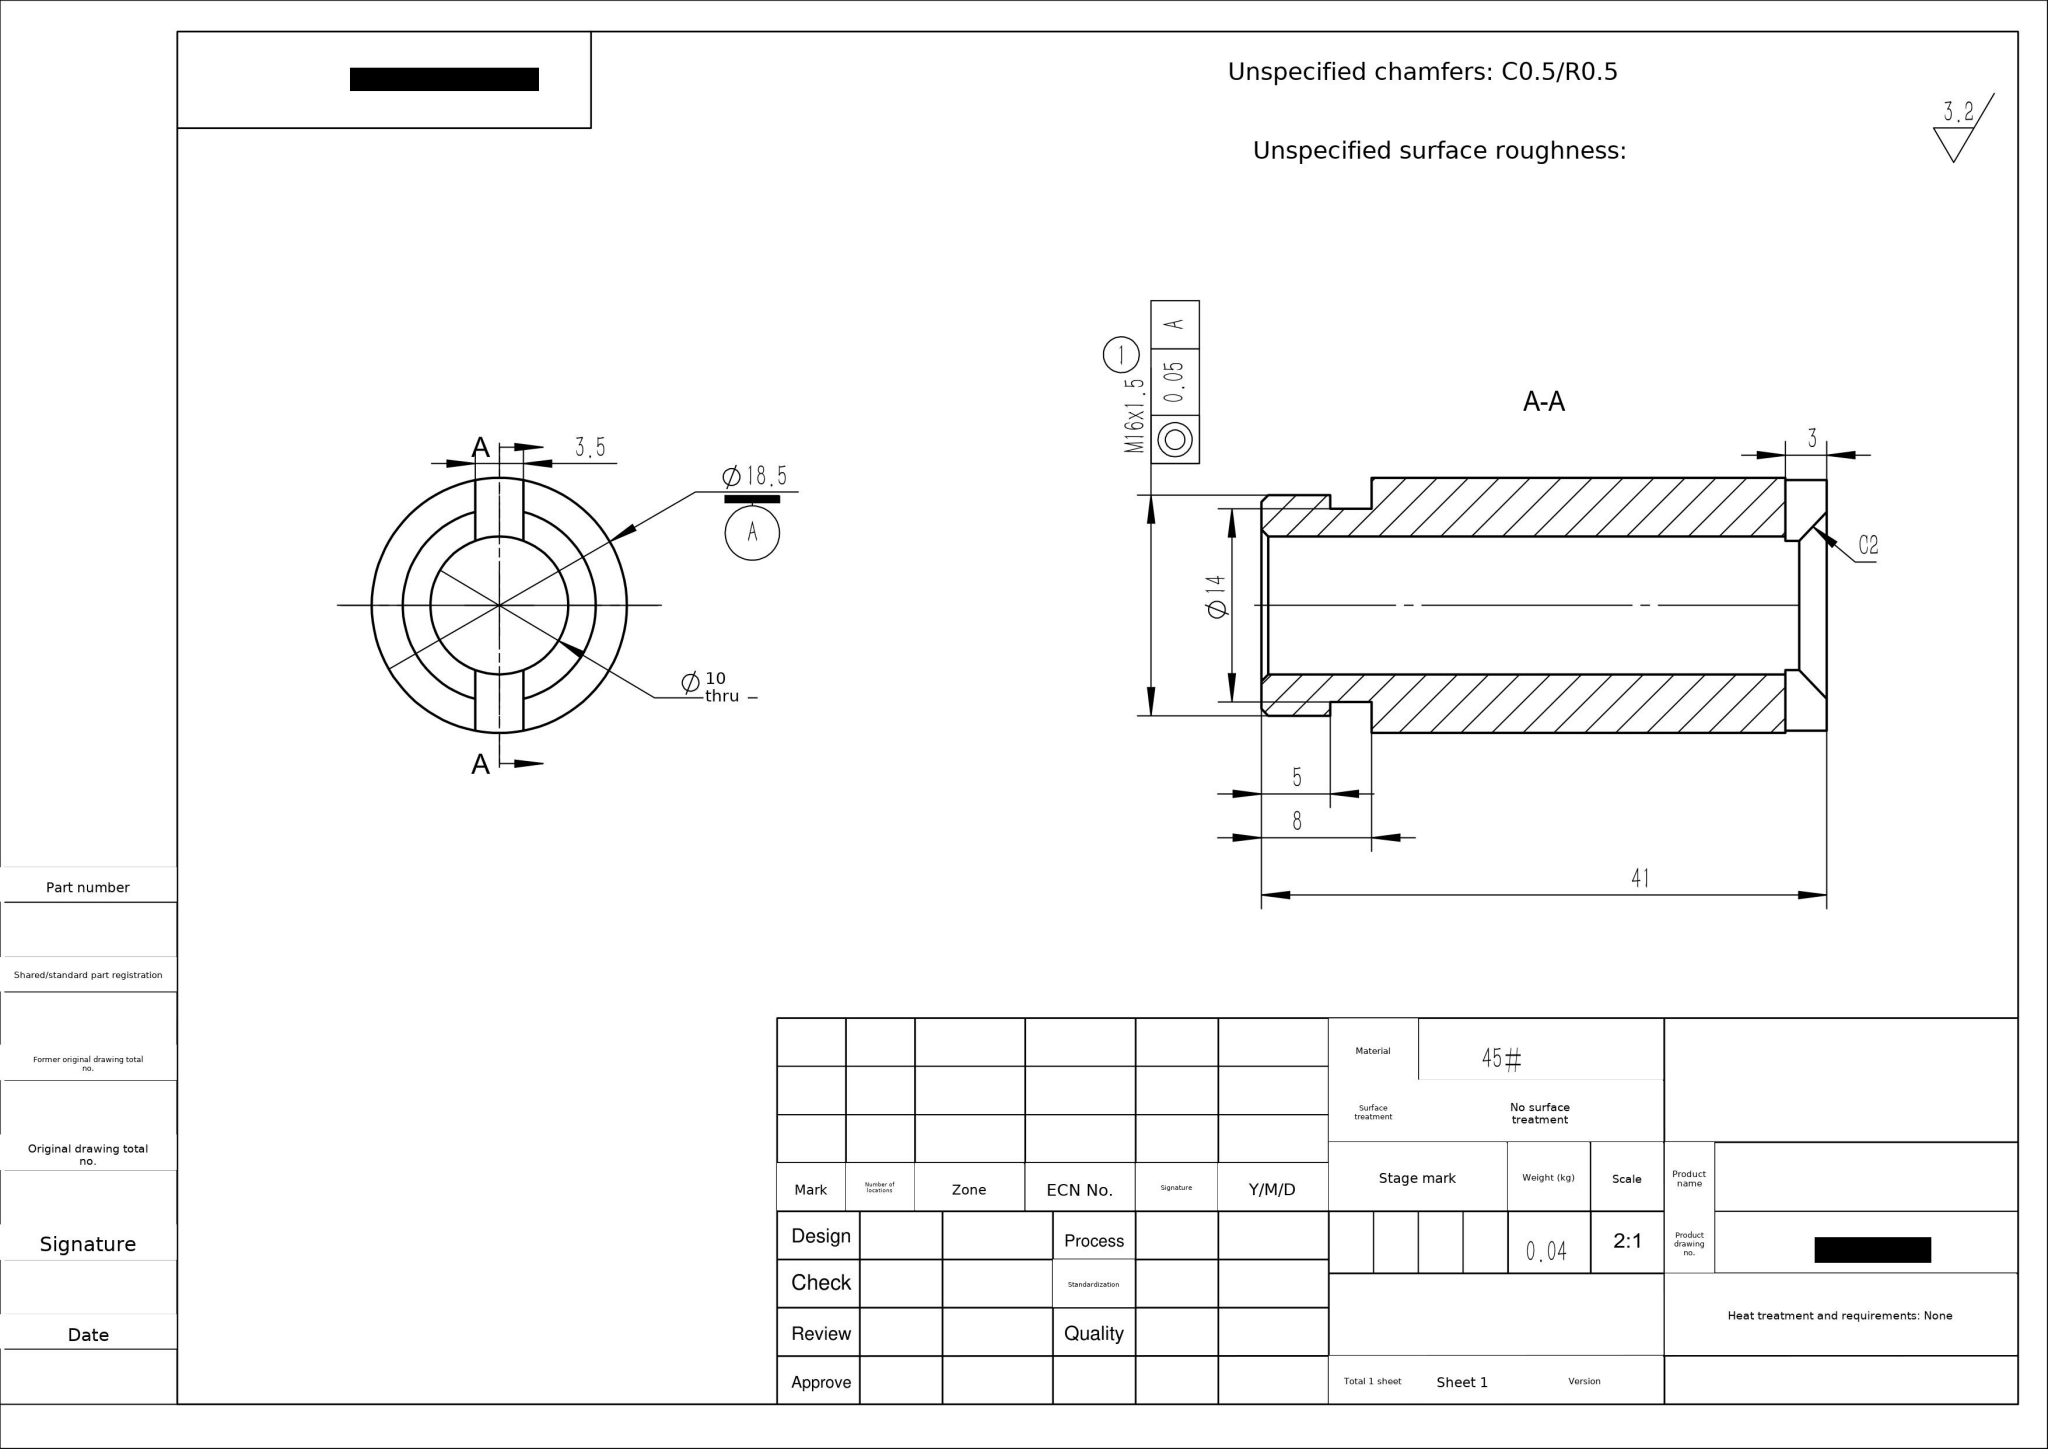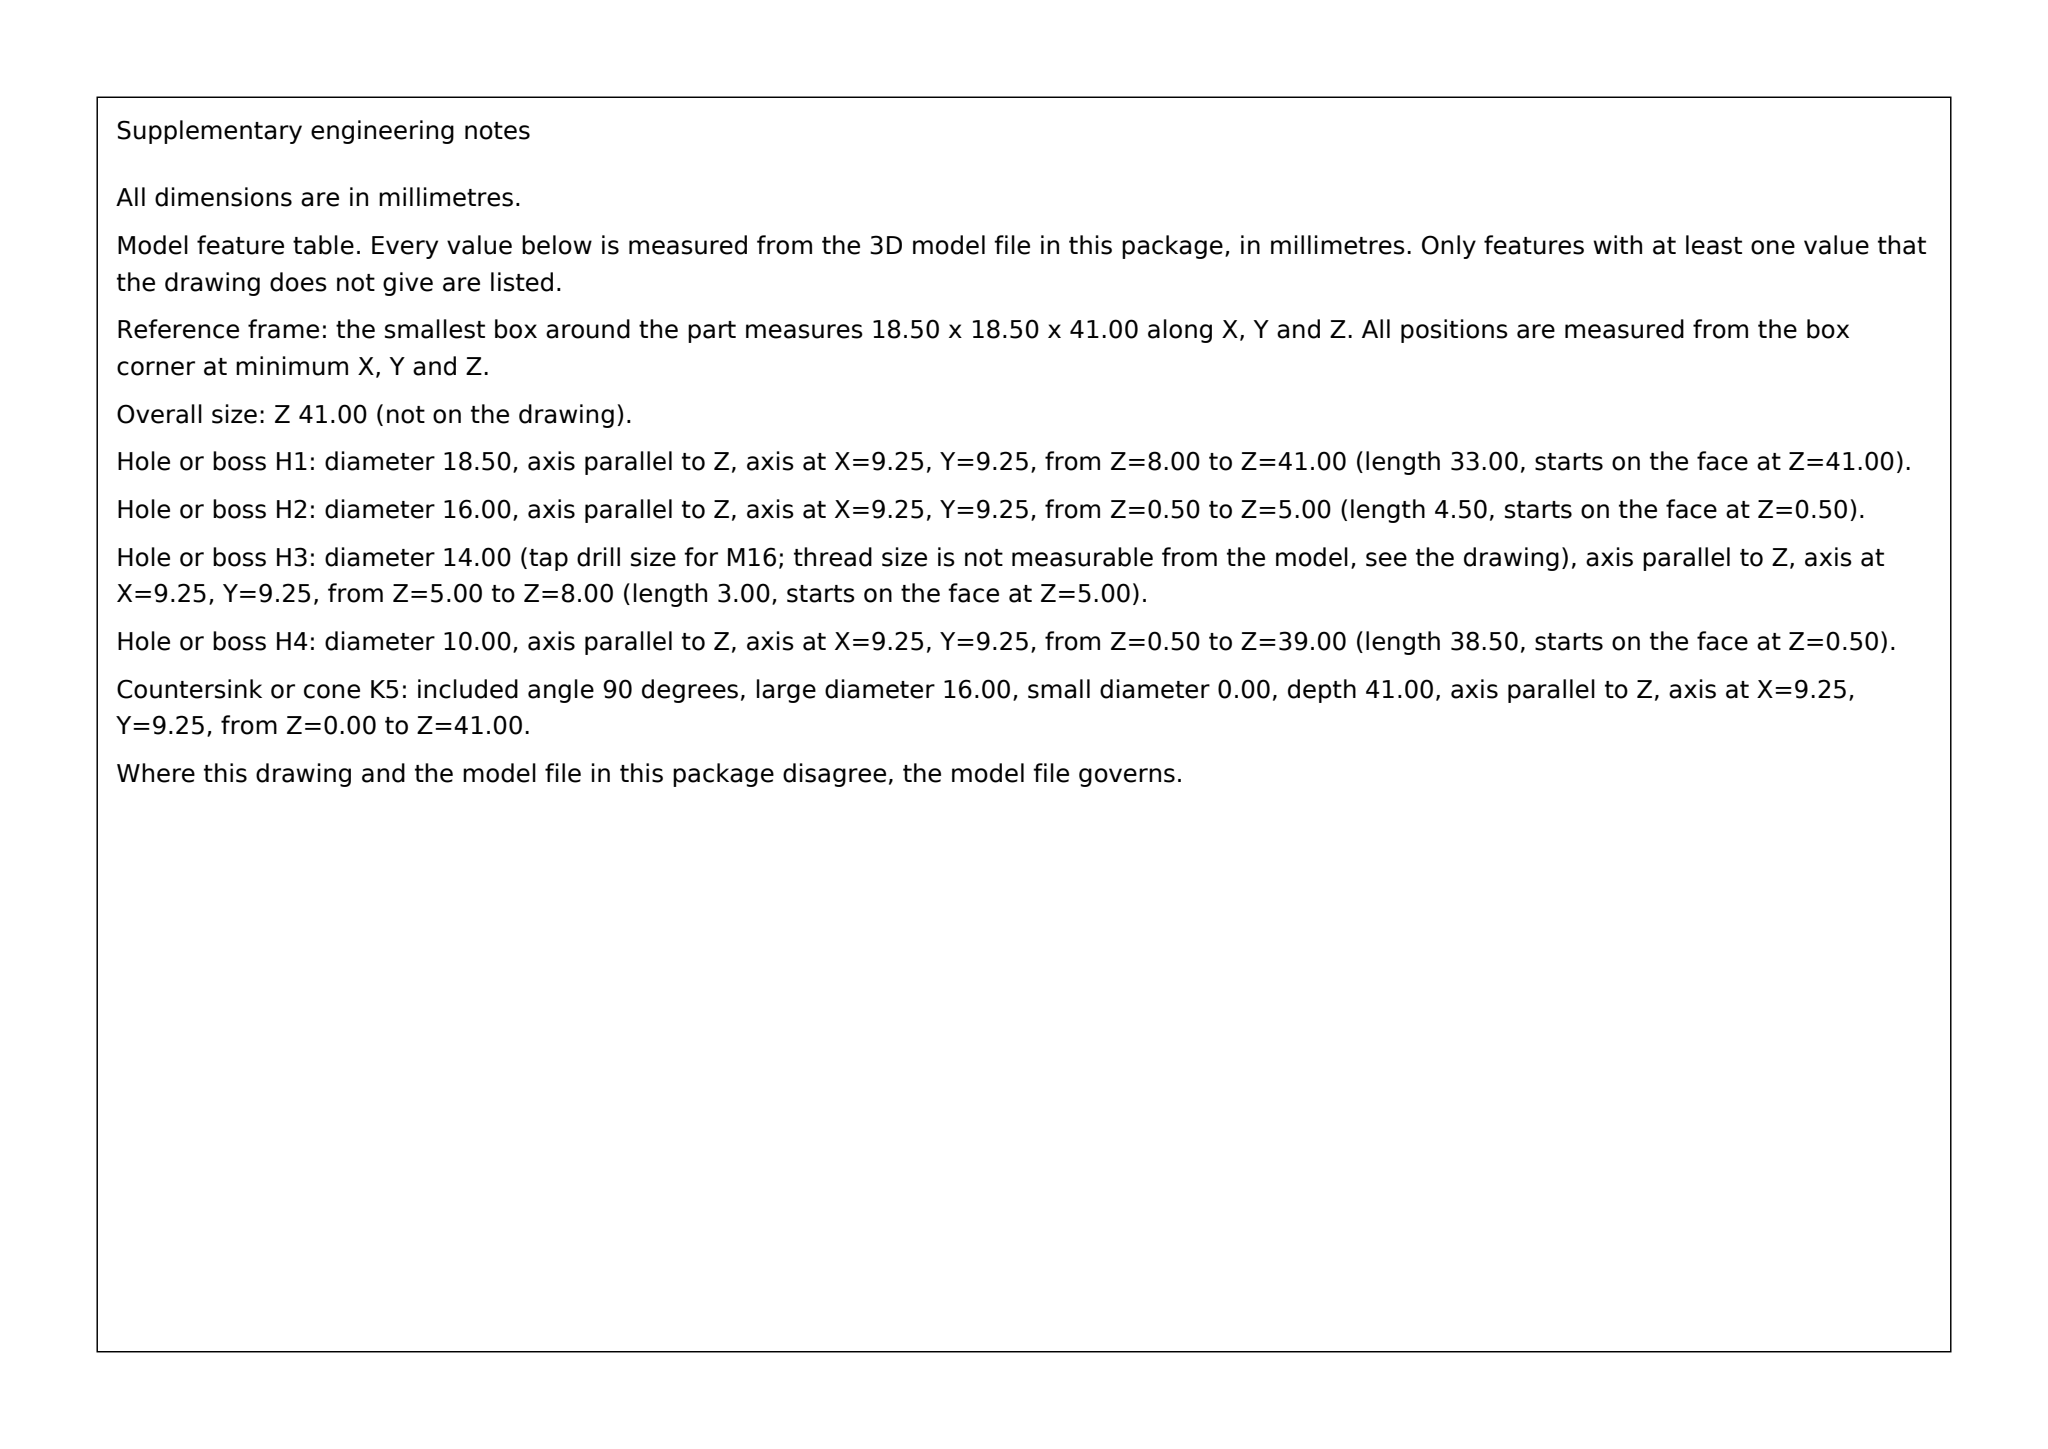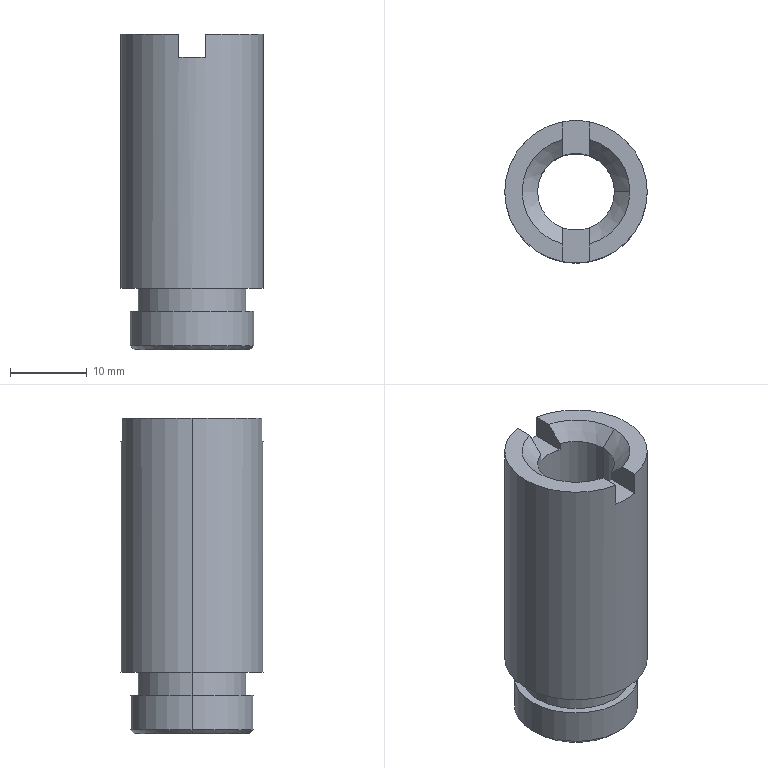Part | SolidWorks | mm | material 45# | 1 solid | 26 faces | box 18.5 x 18.5 x 41 mm | volume 6960 mm3 | plane 11 | cylinder 8 | cone 7 | commonest cylinder face diameters 14 x2 16 x2 10 x2 18.5 x2
STEP:
#1=CARTESIAN_POINT('',(-7.,0.,-3.));
#2=VERTEX_POINT('',#1);
#3=CARTESIAN_POINT('',(7.,0.,-3.));
#4=VERTEX_POINT('',#3);
#5=CARTESIAN_POINT('',(0.,0.,-3.));
#6=DIRECTION('',(0.,0.,-1.));
#7=DIRECTION('',(-1.,0.,0.));
#8=AXIS2_PLACEMENT_3D('',#5,#6,#7);
#9=CIRCLE('',#8,7.);
#10=EDGE_CURVE('',#2,#4,#9,.T.);
#11=ORIENTED_EDGE('',*,*,#10,.F.);
#12=CARTESIAN_POINT('',(-7.,0.,0.));
#13=VERTEX_POINT('',#12);
#14=CARTESIAN_POINT('',(-7.,0.,-3.));
#15=DIRECTION('',(0.,0.,1.));
#16=VECTOR('',#15,1000.);
#17=LINE('',#14,#16);
#18=EDGE_CURVE('',#2,#13,#17,.T.);
#19=ORIENTED_EDGE('',*,*,#18,.T.);
#20=CARTESIAN_POINT('',(7.,0.,0.));
#21=VERTEX_POINT('',#20);
#22=CARTESIAN_POINT('',(0.,0.,0.));
#23=DIRECTION('',(0.,0.,-1.));
#24=DIRECTION('',(-1.,0.,0.));
#25=AXIS2_PLACEMENT_3D('',#22,#23,#24);
#26=CIRCLE('',#25,7.);
#27=EDGE_CURVE('',#13,#21,#26,.T.);
#28=ORIENTED_EDGE('',*,*,#27,.T.);
#29=CARTESIAN_POINT('',(7.,0.,-3.));
#30=DIRECTION('',(0.,0.,1.));
#31=VECTOR('',#30,1000.);
#32=LINE('',#29,#31);
#33=EDGE_CURVE('',#4,#21,#32,.T.);
#34=ORIENTED_EDGE('',*,*,#33,.F.);
#35=EDGE_LOOP('',(#11,#19,#28,#34));
#36=FACE_OUTER_BOUND('',#35,.T.);
#37=CARTESIAN_POINT('',(0.,0.,-3.));
#38=DIRECTION('',(0.,0.,1.));
#39=DIRECTION('',(1.,0.,0.));
#40=AXIS2_PLACEMENT_3D('',#37,#38,#39);
#41=CYLINDRICAL_SURFACE('',#40,7.);
#42=ADVANCED_FACE('',(#36),#41,.T.);
#43=CARTESIAN_POINT('',(-7.5,0.,-8.));
#44=VERTEX_POINT('',#43);
#45=CARTESIAN_POINT('',(7.5,0.,-8.));
#46=VERTEX_POINT('',#45);
#47=CARTESIAN_POINT('',(0.,0.,-8.));
#48=DIRECTION('',(0.,0.,-1.));
#49=DIRECTION('',(-1.,0.,0.));
#50=AXIS2_PLACEMENT_3D('',#47,#48,#49);
#51=CIRCLE('',#50,7.5);
#52=EDGE_CURVE('',#44,#46,#51,.T.);
#53=ORIENTED_EDGE('',*,*,#52,.F.);
#54=CARTESIAN_POINT('',(-8.,0.,-7.5));
#55=VERTEX_POINT('',#54);
#56=CARTESIAN_POINT('',(-7.5,0.,-8.));
#57=DIRECTION('',(-0.7071,0.,0.7071));
#58=VECTOR('',#57,1000.);
#59=LINE('',#56,#58);
#60=EDGE_CURVE('',#44,#55,#59,.T.);
#61=ORIENTED_EDGE('',*,*,#60,.T.);
#62=CARTESIAN_POINT('',(8.,0.,-7.5));
#63=VERTEX_POINT('',#62);
#64=CARTESIAN_POINT('',(0.,0.,-7.5));
#65=DIRECTION('',(0.,0.,1.));
#66=DIRECTION('',(-1.,0.,0.));
#67=AXIS2_PLACEMENT_3D('',#64,#65,#66);
#68=CIRCLE('',#67,8.);
#69=EDGE_CURVE('',#63,#55,#68,.T.);
#70=ORIENTED_EDGE('',*,*,#69,.F.);
#71=CARTESIAN_POINT('',(7.5,0.,-8.));
#72=DIRECTION('',(0.7071,0.,0.7071));
#73=VECTOR('',#72,1000.);
#74=LINE('',#71,#73);
#75=EDGE_CURVE('',#46,#63,#74,.T.);
#76=ORIENTED_EDGE('',*,*,#75,.F.);
#77=EDGE_LOOP('',(#53,#61,#70,#76));
#78=FACE_OUTER_BOUND('',#77,.T.);
#79=CARTESIAN_POINT('',(0.,0.,-8.));
#80=DIRECTION('',(0.,0.,1.));
#81=DIRECTION('',(1.,0.,0.));
#82=AXIS2_PLACEMENT_3D('',#79,#80,#81);
#83=CONICAL_SURFACE('',#82,7.5,0.7854);
#84=ADVANCED_FACE('',(#78),#83,.T.);
#85=CARTESIAN_POINT('',(5.,0.,-7.5));
#86=VERTEX_POINT('',#85);
#87=CARTESIAN_POINT('',(-5.,0.,-7.5));
#88=VERTEX_POINT('',#87);
#89=CARTESIAN_POINT('',(0.,0.,-7.5));
#90=DIRECTION('',(0.,0.,-1.));
#91=DIRECTION('',(-1.,0.,0.));
#92=AXIS2_PLACEMENT_3D('',#89,#90,#91);
#93=CIRCLE('',#92,5.);
#94=EDGE_CURVE('',#86,#88,#93,.T.);
#95=ORIENTED_EDGE('',*,*,#94,.F.);
#96=CARTESIAN_POINT('',(5.5,0.,-8.));
#97=VERTEX_POINT('',#96);
#98=CARTESIAN_POINT('',(5.,0.,-7.5));
#99=DIRECTION('',(0.7071,0.,-0.7071));
#100=VECTOR('',#99,1000.);
#101=LINE('',#98,#100);
#102=EDGE_CURVE('',#86,#97,#101,.T.);
#103=ORIENTED_EDGE('',*,*,#102,.T.);
#104=CARTESIAN_POINT('',(-5.5,0.,-8.));
#105=VERTEX_POINT('',#104);
#106=CARTESIAN_POINT('',(0.,0.,-8.));
#107=DIRECTION('',(0.,0.,1.));
#108=DIRECTION('',(-1.,0.,0.));
#109=AXIS2_PLACEMENT_3D('',#106,#107,#108);
#110=CIRCLE('',#109,5.5);
#111=EDGE_CURVE('',#105,#97,#110,.T.);
#112=ORIENTED_EDGE('',*,*,#111,.F.);
#113=CARTESIAN_POINT('',(-5.,0.,-7.5));
#114=DIRECTION('',(-0.7071,0.,-0.7071));
#115=VECTOR('',#114,1000.);
#116=LINE('',#113,#115);
#117=EDGE_CURVE('',#88,#105,#116,.T.);
#118=ORIENTED_EDGE('',*,*,#117,.F.);
#119=EDGE_LOOP('',(#95,#103,#112,#118));
#120=FACE_OUTER_BOUND('',#119,.T.);
#121=CARTESIAN_POINT('',(0.,0.,-7.5));
#122=DIRECTION('',(0.,0.,-1.));
#123=DIRECTION('',(-1.,0.,0.));
#124=AXIS2_PLACEMENT_3D('',#121,#122,#123);
#125=CONICAL_SURFACE('',#124,5.,0.7854);
#126=ADVANCED_FACE('',(#120),#125,.F.);
#127=ORIENTED_EDGE('',*,*,#69,.T.);
#128=CARTESIAN_POINT('',(-8.,0.,-3.));
#129=VERTEX_POINT('',#128);
#130=CARTESIAN_POINT('',(-8.,0.,-8.));
#131=DIRECTION('',(0.,0.,1.));
#132=VECTOR('',#131,1000.);
#133=LINE('',#130,#132);
#134=EDGE_CURVE('',#55,#129,#133,.T.);
#135=ORIENTED_EDGE('',*,*,#134,.T.);
#136=CARTESIAN_POINT('',(8.,0.,-3.));
#137=VERTEX_POINT('',#136);
#138=CARTESIAN_POINT('',(0.,0.,-3.));
#139=DIRECTION('',(0.,0.,-1.));
#140=DIRECTION('',(-1.,0.,0.));
#141=AXIS2_PLACEMENT_3D('',#138,#139,#140);
#142=CIRCLE('',#141,8.);
#143=EDGE_CURVE('',#129,#137,#142,.T.);
#144=ORIENTED_EDGE('',*,*,#143,.T.);
#145=CARTESIAN_POINT('',(8.,0.,-8.));
#146=DIRECTION('',(0.,0.,1.));
#147=VECTOR('',#146,1000.);
#148=LINE('',#145,#147);
#149=EDGE_CURVE('',#63,#137,#148,.T.);
#150=ORIENTED_EDGE('',*,*,#149,.F.);
#151=EDGE_LOOP('',(#127,#135,#144,#150));
#152=FACE_OUTER_BOUND('',#151,.T.);
#153=CARTESIAN_POINT('',(0.,0.,-8.));
#154=DIRECTION('',(0.,0.,1.));
#155=DIRECTION('',(1.,0.,0.));
#156=AXIS2_PLACEMENT_3D('',#153,#154,#155);
#157=CYLINDRICAL_SURFACE('',#156,8.);
#158=ADVANCED_FACE('',(#152),#157,.T.);
#159=CARTESIAN_POINT('',(1.75,-4.684,31.));
#160=VERTEX_POINT('',#159);
#161=CARTESIAN_POINT('',(5.,0.,31.));
#162=VERTEX_POINT('',#161);
#163=CARTESIAN_POINT('',(0.,0.,31.));
#164=DIRECTION('',(0.,0.,1.));
#165=DIRECTION('',(1.,0.,0.));
#166=AXIS2_PLACEMENT_3D('',#163,#164,#165);
#167=CIRCLE('',#166,5.);
#168=EDGE_CURVE('',#160,#162,#167,.T.);
#169=ORIENTED_EDGE('',*,*,#168,.T.);
#170=CARTESIAN_POINT('',(5.,0.,33.));
#171=DIRECTION('',(0.,0.,-1.));
#172=VECTOR('',#171,1000.);
#173=LINE('',#170,#172);
#174=EDGE_CURVE('',#162,#86,#173,.T.);
#175=ORIENTED_EDGE('',*,*,#174,.T.);
#176=ORIENTED_EDGE('',*,*,#94,.T.);
#177=CARTESIAN_POINT('',(-5.,0.,31.));
#178=VERTEX_POINT('',#177);
#179=CARTESIAN_POINT('',(-5.,0.,33.));
#180=DIRECTION('',(0.,0.,-1.));
#181=VECTOR('',#180,1000.);
#182=LINE('',#179,#181);
#183=EDGE_CURVE('',#178,#88,#182,.T.);
#184=ORIENTED_EDGE('',*,*,#183,.F.);
#185=CARTESIAN_POINT('',(-1.75,-4.684,31.));
#186=VERTEX_POINT('',#185);
#187=CARTESIAN_POINT('',(0.,0.,31.));
#188=DIRECTION('',(0.,0.,1.));
#189=DIRECTION('',(1.,0.,0.));
#190=AXIS2_PLACEMENT_3D('',#187,#188,#189);
#191=CIRCLE('',#190,5.);
#192=EDGE_CURVE('',#178,#186,#191,.T.);
#193=ORIENTED_EDGE('',*,*,#192,.T.);
#194=CARTESIAN_POINT('',(-1.75,-4.684,30.));
#195=VERTEX_POINT('',#194);
#196=CARTESIAN_POINT('',(-1.75,-4.684,33.));
#197=DIRECTION('',(0.,0.,1.));
#198=VECTOR('',#197,1000.);
#199=LINE('',#196,#198);
#200=EDGE_CURVE('',#195,#186,#199,.T.);
#201=ORIENTED_EDGE('',*,*,#200,.F.);
#202=CARTESIAN_POINT('',(1.75,-4.684,30.));
#203=VERTEX_POINT('',#202);
#204=CARTESIAN_POINT('',(0.,0.,30.));
#205=DIRECTION('',(0.,0.,1.));
#206=DIRECTION('',(1.,0.,0.));
#207=AXIS2_PLACEMENT_3D('',#204,#205,#206);
#208=CIRCLE('',#207,5.);
#209=EDGE_CURVE('',#195,#203,#208,.T.);
#210=ORIENTED_EDGE('',*,*,#209,.T.);
#211=CARTESIAN_POINT('',(1.75,-4.684,33.));
#212=DIRECTION('',(0.,0.,-1.));
#213=VECTOR('',#212,1000.);
#214=LINE('',#211,#213);
#215=EDGE_CURVE('',#160,#203,#214,.T.);
#216=ORIENTED_EDGE('',*,*,#215,.F.);
#217=EDGE_LOOP('',(#169,#175,#176,#184,#193,#201,#210,#216));
#218=FACE_OUTER_BOUND('',#217,.T.);
#219=CARTESIAN_POINT('',(0.,0.,33.));
#220=DIRECTION('',(0.,0.,-1.));
#221=DIRECTION('',(-1.,0.,0.));
#222=AXIS2_PLACEMENT_3D('',#219,#220,#221);
#223=CYLINDRICAL_SURFACE('',#222,5.);
#224=ADVANCED_FACE('',(#218),#223,.F.);
#225=CARTESIAN_POINT('',(9.25,0.,33.));
#226=VERTEX_POINT('',#225);
#227=CARTESIAN_POINT('',(1.75,9.083,33.));
#228=VERTEX_POINT('',#227);
#229=CARTESIAN_POINT('',(0.,0.,33.));
#230=DIRECTION('',(0.,0.,1.));
#231=DIRECTION('',(1.,0.,0.));
#232=AXIS2_PLACEMENT_3D('',#229,#230,#231);
#233=CIRCLE('',#232,9.25);
#234=EDGE_CURVE('',#226,#228,#233,.T.);
#235=ORIENTED_EDGE('',*,*,#234,.F.);
#236=CARTESIAN_POINT('',(9.25,0.,0.));
#237=VERTEX_POINT('',#236);
#238=CARTESIAN_POINT('',(9.25,0.,33.));
#239=DIRECTION('',(0.,0.,-1.));
#240=VECTOR('',#239,1000.);
#241=LINE('',#238,#240);
#242=EDGE_CURVE('',#226,#237,#241,.T.);
#243=ORIENTED_EDGE('',*,*,#242,.T.);
#244=CARTESIAN_POINT('',(-9.25,0.,0.));
#245=VERTEX_POINT('',#244);
#246=CARTESIAN_POINT('',(0.,0.,0.));
#247=DIRECTION('',(0.,0.,1.));
#248=DIRECTION('',(1.,0.,0.));
#249=AXIS2_PLACEMENT_3D('',#246,#247,#248);
#250=CIRCLE('',#249,9.25);
#251=EDGE_CURVE('',#237,#245,#250,.T.);
#252=ORIENTED_EDGE('',*,*,#251,.T.);
#253=CARTESIAN_POINT('',(-9.25,0.,33.));
#254=VERTEX_POINT('',#253);
#255=CARTESIAN_POINT('',(-9.25,0.,33.));
#256=DIRECTION('',(0.,0.,-1.));
#257=VECTOR('',#256,1000.);
#258=LINE('',#255,#257);
#259=EDGE_CURVE('',#254,#245,#258,.T.);
#260=ORIENTED_EDGE('',*,*,#259,.F.);
#261=CARTESIAN_POINT('',(-1.75,9.083,33.));
#262=VERTEX_POINT('',#261);
#263=CARTESIAN_POINT('',(0.,0.,33.));
#264=DIRECTION('',(0.,0.,1.));
#265=DIRECTION('',(1.,0.,0.));
#266=AXIS2_PLACEMENT_3D('',#263,#264,#265);
#267=CIRCLE('',#266,9.25);
#268=EDGE_CURVE('',#262,#254,#267,.T.);
#269=ORIENTED_EDGE('',*,*,#268,.F.);
#270=CARTESIAN_POINT('',(-1.75,9.083,30.));
#271=VERTEX_POINT('',#270);
#272=CARTESIAN_POINT('',(-1.75,9.083,33.));
#273=DIRECTION('',(0.,0.,-1.));
#274=VECTOR('',#273,1000.);
#275=LINE('',#272,#274);
#276=EDGE_CURVE('',#262,#271,#275,.T.);
#277=ORIENTED_EDGE('',*,*,#276,.T.);
#278=CARTESIAN_POINT('',(1.75,9.083,30.));
#279=VERTEX_POINT('',#278);
#280=CARTESIAN_POINT('',(0.,0.,30.));
#281=DIRECTION('',(0.,0.,1.));
#282=DIRECTION('',(1.,0.,0.));
#283=AXIS2_PLACEMENT_3D('',#280,#281,#282);
#284=CIRCLE('',#283,9.25);
#285=EDGE_CURVE('',#279,#271,#284,.T.);
#286=ORIENTED_EDGE('',*,*,#285,.F.);
#287=CARTESIAN_POINT('',(1.75,9.083,33.));
#288=DIRECTION('',(0.,0.,1.));
#289=VECTOR('',#288,1000.);
#290=LINE('',#287,#289);
#291=EDGE_CURVE('',#279,#228,#290,.T.);
#292=ORIENTED_EDGE('',*,*,#291,.T.);
#293=EDGE_LOOP('',(#235,#243,#252,#260,#269,#277,#286,#292));
#294=FACE_OUTER_BOUND('',#293,.T.);
#295=CARTESIAN_POINT('',(0.,0.,33.));
#296=DIRECTION('',(0.,0.,-1.));
#297=DIRECTION('',(-1.,0.,0.));
#298=AXIS2_PLACEMENT_3D('',#295,#296,#297);
#299=CYLINDRICAL_SURFACE('',#298,9.25);
#300=ADVANCED_FACE('',(#294),#299,.T.);
#301=CARTESIAN_POINT('',(1.75,4.684,31.));
#302=VERTEX_POINT('',#301);
#303=CARTESIAN_POINT('',(0.,0.,31.));
#304=DIRECTION('',(0.,0.,1.));
#305=DIRECTION('',(1.,0.,0.));
#306=AXIS2_PLACEMENT_3D('',#303,#304,#305);
#307=CIRCLE('',#306,5.);
#308=EDGE_CURVE('',#162,#302,#307,.T.);
#309=ORIENTED_EDGE('',*,*,#308,.F.);
#310=CARTESIAN_POINT('',(7.,0.,33.));
#311=VERTEX_POINT('',#310);
#312=CARTESIAN_POINT('',(5.,0.,31.));
#313=DIRECTION('',(0.7071,0.,0.7071));
#314=VECTOR('',#313,1000.);
#315=LINE('',#312,#314);
#316=EDGE_CURVE('',#162,#311,#315,.T.);
#317=ORIENTED_EDGE('',*,*,#316,.T.);
#318=CARTESIAN_POINT('',(1.75,6.778,33.));
#319=VERTEX_POINT('',#318);
#320=CARTESIAN_POINT('',(0.,0.,33.));
#321=DIRECTION('',(0.,0.,-1.));
#322=DIRECTION('',(1.,0.,0.));
#323=AXIS2_PLACEMENT_3D('',#320,#321,#322);
#324=CIRCLE('',#323,7.);
#325=EDGE_CURVE('',#319,#311,#324,.T.);
#326=ORIENTED_EDGE('',*,*,#325,.F.);
#327=CARTESIAN_POINT('',(1.75,4.684,31.));
#328=CARTESIAN_POINT('',(1.75,5.388,31.66));
#329=CARTESIAN_POINT('',(1.75,6.084,32.328));
#330=CARTESIAN_POINT('',(1.75,6.778,33.));
#331=B_SPLINE_CURVE_WITH_KNOTS('',3,(#327,#328,#329,#330),.UNSPECIFIED.,.F.,.F.,(4,4),(0.02649,0.02936),.UNSPECIFIED.);
#332=EDGE_CURVE('',#302,#319,#331,.T.);
#333=ORIENTED_EDGE('',*,*,#332,.F.);
#334=EDGE_LOOP('',(#309,#317,#326,#333));
#335=FACE_OUTER_BOUND('',#334,.T.);
#336=CARTESIAN_POINT('',(0.,0.,31.));
#337=DIRECTION('',(0.,0.,1.));
#338=DIRECTION('',(1.,0.,0.));
#339=AXIS2_PLACEMENT_3D('',#336,#337,#338);
#340=CONICAL_SURFACE('',#339,5.,0.7854);
#341=ADVANCED_FACE('',(#335),#340,.F.);
#342=CARTESIAN_POINT('',(1.75,-9.083,33.));
#343=VERTEX_POINT('',#342);
#344=CARTESIAN_POINT('',(1.75,-6.778,33.));
#345=VERTEX_POINT('',#344);
#346=CARTESIAN_POINT('',(1.75,15.,33.));
#347=DIRECTION('',(-0.,1.,0.));
#348=VECTOR('',#347,1000.);
#349=LINE('',#346,#348);
#350=EDGE_CURVE('',#343,#345,#349,.T.);
#351=ORIENTED_EDGE('',*,*,#350,.F.);
#352=CARTESIAN_POINT('',(0.,0.,33.));
#353=DIRECTION('',(0.,0.,1.));
#354=DIRECTION('',(1.,0.,0.));
#355=AXIS2_PLACEMENT_3D('',#352,#353,#354);
#356=CIRCLE('',#355,9.25);
#357=EDGE_CURVE('',#343,#226,#356,.T.);
#358=ORIENTED_EDGE('',*,*,#357,.T.);
#359=ORIENTED_EDGE('',*,*,#234,.T.);
#360=CARTESIAN_POINT('',(1.75,15.,33.));
#361=DIRECTION('',(-0.,1.,0.));
#362=VECTOR('',#361,1000.);
#363=LINE('',#360,#362);
#364=EDGE_CURVE('',#319,#228,#363,.T.);
#365=ORIENTED_EDGE('',*,*,#364,.F.);
#366=ORIENTED_EDGE('',*,*,#325,.T.);
#367=CARTESIAN_POINT('',(0.,0.,33.));
#368=DIRECTION('',(0.,0.,-1.));
#369=DIRECTION('',(1.,0.,0.));
#370=AXIS2_PLACEMENT_3D('',#367,#368,#369);
#371=CIRCLE('',#370,7.);
#372=EDGE_CURVE('',#311,#345,#371,.T.);
#373=ORIENTED_EDGE('',*,*,#372,.T.);
#374=EDGE_LOOP('',(#351,#358,#359,#365,#366,#373));
#375=FACE_OUTER_BOUND('',#374,.T.);
#376=CARTESIAN_POINT('',(0.,0.,33.));
#377=DIRECTION('',(0.,0.,1.));
#378=DIRECTION('',(1.,0.,0.));
#379=AXIS2_PLACEMENT_3D('',#376,#377,#378);
#380=PLANE('',#379);
#381=ADVANCED_FACE('',(#375),#380,.T.);
#382=ORIENTED_EDGE('',*,*,#316,.F.);
#383=ORIENTED_EDGE('',*,*,#168,.F.);
#384=CARTESIAN_POINT('',(1.75,-6.778,33.));
#385=CARTESIAN_POINT('',(1.75,-6.084,32.329));
#386=CARTESIAN_POINT('',(1.75,-5.388,31.66));
#387=CARTESIAN_POINT('',(1.75,-4.684,31.));
#388=B_SPLINE_CURVE_WITH_KNOTS('',3,(#384,#385,#386,#387),.UNSPECIFIED.,.F.,.F.,(4,4),(0.01209,0.01498),.UNSPECIFIED.);
#389=EDGE_CURVE('',#345,#160,#388,.T.);
#390=ORIENTED_EDGE('',*,*,#389,.F.);
#391=ORIENTED_EDGE('',*,*,#372,.F.);
#392=EDGE_LOOP('',(#382,#383,#390,#391));
#393=FACE_OUTER_BOUND('',#392,.T.);
#394=CARTESIAN_POINT('',(0.,0.,31.));
#395=DIRECTION('',(0.,0.,1.));
#396=DIRECTION('',(1.,0.,0.));
#397=AXIS2_PLACEMENT_3D('',#394,#395,#396);
#398=CONICAL_SURFACE('',#397,5.,0.7854);
#399=ADVANCED_FACE('',(#393),#398,.F.);
#400=CARTESIAN_POINT('',(-1.75,6.778,33.));
#401=VERTEX_POINT('',#400);
#402=CARTESIAN_POINT('',(-1.75,15.,33.));
#403=DIRECTION('',(0.,-1.,0.));
#404=VECTOR('',#403,1000.);
#405=LINE('',#402,#404);
#406=EDGE_CURVE('',#262,#401,#405,.T.);
#407=ORIENTED_EDGE('',*,*,#406,.F.);
#408=ORIENTED_EDGE('',*,*,#268,.T.);
#409=CARTESIAN_POINT('',(-1.75,-9.083,33.));
#410=VERTEX_POINT('',#409);
#411=CARTESIAN_POINT('',(0.,0.,33.));
#412=DIRECTION('',(0.,0.,1.));
#413=DIRECTION('',(1.,0.,0.));
#414=AXIS2_PLACEMENT_3D('',#411,#412,#413);
#415=CIRCLE('',#414,9.25);
#416=EDGE_CURVE('',#254,#410,#415,.T.);
#417=ORIENTED_EDGE('',*,*,#416,.T.);
#418=CARTESIAN_POINT('',(-1.75,-6.778,33.));
#419=VERTEX_POINT('',#418);
#420=CARTESIAN_POINT('',(-1.75,15.,33.));
#421=DIRECTION('',(0.,-1.,0.));
#422=VECTOR('',#421,1000.);
#423=LINE('',#420,#422);
#424=EDGE_CURVE('',#419,#410,#423,.T.);
#425=ORIENTED_EDGE('',*,*,#424,.F.);
#426=CARTESIAN_POINT('',(0.,0.,33.));
#427=DIRECTION('',(0.,0.,-1.));
#428=DIRECTION('',(1.,0.,0.));
#429=AXIS2_PLACEMENT_3D('',#426,#427,#428);
#430=CIRCLE('',#429,7.);
#431=EDGE_CURVE('',#419,#401,#430,.T.);
#432=ORIENTED_EDGE('',*,*,#431,.T.);
#433=EDGE_LOOP('',(#407,#408,#417,#425,#432));
#434=FACE_OUTER_BOUND('',#433,.T.);
#435=CARTESIAN_POINT('',(0.,0.,33.));
#436=DIRECTION('',(0.,0.,1.));
#437=DIRECTION('',(1.,0.,0.));
#438=AXIS2_PLACEMENT_3D('',#435,#436,#437);
#439=PLANE('',#438);
#440=ADVANCED_FACE('',(#434),#439,.T.);
#441=CARTESIAN_POINT('',(0.,0.,0.));
#442=DIRECTION('',(0.,0.,1.));
#443=DIRECTION('',(1.,0.,0.));
#444=AXIS2_PLACEMENT_3D('',#441,#442,#443);
#445=CIRCLE('',#444,9.25);
#446=EDGE_CURVE('',#245,#237,#445,.T.);
#447=ORIENTED_EDGE('',*,*,#446,.F.);
#448=ORIENTED_EDGE('',*,*,#251,.F.);
#449=EDGE_LOOP('',(#447,#448));
#450=FACE_OUTER_BOUND('',#449,.T.);
#451=CARTESIAN_POINT('',(0.,0.,0.));
#452=DIRECTION('',(0.,0.,-1.));
#453=DIRECTION('',(-1.,0.,0.));
#454=AXIS2_PLACEMENT_3D('',#451,#452,#453);
#455=CIRCLE('',#454,7.);
#456=EDGE_CURVE('',#21,#13,#455,.T.);
#457=ORIENTED_EDGE('',*,*,#456,.F.);
#458=ORIENTED_EDGE('',*,*,#27,.F.);
#459=EDGE_LOOP('',(#457,#458));
#460=FACE_BOUND('',#459,.T.);
#461=CARTESIAN_POINT('',(0.,0.,0.));
#462=DIRECTION('',(0.,0.,1.));
#463=DIRECTION('',(1.,0.,0.));
#464=AXIS2_PLACEMENT_3D('',#461,#462,#463);
#465=PLANE('',#464);
#466=ADVANCED_FACE('',(#450,#460),#465,.F.);
#467=ORIENTED_EDGE('',*,*,#242,.F.);
#468=ORIENTED_EDGE('',*,*,#357,.F.);
#469=CARTESIAN_POINT('',(1.75,-9.083,30.));
#470=VERTEX_POINT('',#469);
#471=CARTESIAN_POINT('',(1.75,-9.083,33.));
#472=DIRECTION('',(0.,0.,-1.));
#473=VECTOR('',#472,1000.);
#474=LINE('',#471,#473);
#475=EDGE_CURVE('',#343,#470,#474,.T.);
#476=ORIENTED_EDGE('',*,*,#475,.T.);
#477=CARTESIAN_POINT('',(-1.75,-9.083,30.));
#478=VERTEX_POINT('',#477);
#479=CARTESIAN_POINT('',(0.,0.,30.));
#480=DIRECTION('',(0.,0.,1.));
#481=DIRECTION('',(1.,0.,0.));
#482=AXIS2_PLACEMENT_3D('',#479,#480,#481);
#483=CIRCLE('',#482,9.25);
#484=EDGE_CURVE('',#478,#470,#483,.T.);
#485=ORIENTED_EDGE('',*,*,#484,.F.);
#486=CARTESIAN_POINT('',(-1.75,-9.083,33.));
#487=DIRECTION('',(0.,0.,1.));
#488=VECTOR('',#487,1000.);
#489=LINE('',#486,#488);
#490=EDGE_CURVE('',#478,#410,#489,.T.);
#491=ORIENTED_EDGE('',*,*,#490,.T.);
#492=ORIENTED_EDGE('',*,*,#416,.F.);
#493=ORIENTED_EDGE('',*,*,#259,.T.);
#494=ORIENTED_EDGE('',*,*,#446,.T.);
#495=EDGE_LOOP('',(#467,#468,#476,#485,#491,#492,#493,#494));
#496=FACE_OUTER_BOUND('',#495,.T.);
#497=CARTESIAN_POINT('',(0.,0.,33.));
#498=DIRECTION('',(0.,0.,-1.));
#499=DIRECTION('',(-1.,0.,0.));
#500=AXIS2_PLACEMENT_3D('',#497,#498,#499);
#501=CYLINDRICAL_SURFACE('',#500,9.25);
#502=ADVANCED_FACE('',(#496),#501,.T.);
#503=ORIENTED_EDGE('',*,*,#174,.F.);
#504=ORIENTED_EDGE('',*,*,#308,.T.);
#505=CARTESIAN_POINT('',(1.75,4.684,30.));
#506=VERTEX_POINT('',#505);
#507=CARTESIAN_POINT('',(1.75,4.684,33.));
#508=DIRECTION('',(0.,0.,1.));
#509=VECTOR('',#508,1000.);
#510=LINE('',#507,#509);
#511=EDGE_CURVE('',#506,#302,#510,.T.);
#512=ORIENTED_EDGE('',*,*,#511,.F.);
#513=CARTESIAN_POINT('',(-1.75,4.684,30.));
#514=VERTEX_POINT('',#513);
#515=CARTESIAN_POINT('',(0.,0.,30.));
#516=DIRECTION('',(0.,0.,1.));
#517=DIRECTION('',(1.,0.,0.));
#518=AXIS2_PLACEMENT_3D('',#515,#516,#517);
#519=CIRCLE('',#518,5.);
#520=EDGE_CURVE('',#506,#514,#519,.T.);
#521=ORIENTED_EDGE('',*,*,#520,.T.);
#522=CARTESIAN_POINT('',(-1.75,4.684,31.));
#523=VERTEX_POINT('',#522);
#524=CARTESIAN_POINT('',(-1.75,4.684,33.));
#525=DIRECTION('',(0.,0.,-1.));
#526=VECTOR('',#525,1000.);
#527=LINE('',#524,#526);
#528=EDGE_CURVE('',#523,#514,#527,.T.);
#529=ORIENTED_EDGE('',*,*,#528,.F.);
#530=CARTESIAN_POINT('',(0.,0.,31.));
#531=DIRECTION('',(0.,0.,1.));
#532=DIRECTION('',(1.,0.,0.));
#533=AXIS2_PLACEMENT_3D('',#530,#531,#532);
#534=CIRCLE('',#533,5.);
#535=EDGE_CURVE('',#523,#178,#534,.T.);
#536=ORIENTED_EDGE('',*,*,#535,.T.);
#537=ORIENTED_EDGE('',*,*,#183,.T.);
#538=CARTESIAN_POINT('',(0.,0.,-7.5));
#539=DIRECTION('',(0.,0.,-1.));
#540=DIRECTION('',(-1.,0.,0.));
#541=AXIS2_PLACEMENT_3D('',#538,#539,#540);
#542=CIRCLE('',#541,5.);
#543=EDGE_CURVE('',#88,#86,#542,.T.);
#544=ORIENTED_EDGE('',*,*,#543,.T.);
#545=EDGE_LOOP('',(#503,#504,#512,#521,#529,#536,#537,#544));
#546=FACE_OUTER_BOUND('',#545,.T.);
#547=CARTESIAN_POINT('',(0.,0.,33.));
#548=DIRECTION('',(0.,0.,-1.));
#549=DIRECTION('',(-1.,0.,0.));
#550=AXIS2_PLACEMENT_3D('',#547,#548,#549);
#551=CYLINDRICAL_SURFACE('',#550,5.);
#552=ADVANCED_FACE('',(#546),#551,.F.);
#553=CARTESIAN_POINT('',(-1.75,6.778,33.));
#554=CARTESIAN_POINT('',(-1.75,6.084,32.329));
#555=CARTESIAN_POINT('',(-1.75,5.388,31.66));
#556=CARTESIAN_POINT('',(-1.75,4.684,31.));
#557=B_SPLINE_CURVE_WITH_KNOTS('',3,(#553,#554,#555,#556),.UNSPECIFIED.,.F.,.F.,(4,4),(0.01209,0.01498),.UNSPECIFIED.);
#558=EDGE_CURVE('',#401,#523,#557,.T.);
#559=ORIENTED_EDGE('',*,*,#558,.F.);
#560=ORIENTED_EDGE('',*,*,#431,.F.);
#561=CARTESIAN_POINT('',(-1.75,-4.684,31.));
#562=CARTESIAN_POINT('',(-1.75,-5.388,31.66));
#563=CARTESIAN_POINT('',(-1.75,-6.084,32.328));
#564=CARTESIAN_POINT('',(-1.75,-6.778,33.));
#565=B_SPLINE_CURVE_WITH_KNOTS('',3,(#561,#562,#563,#564),.UNSPECIFIED.,.F.,.F.,(4,4),(0.02649,0.02936),.UNSPECIFIED.);
#566=EDGE_CURVE('',#186,#419,#565,.T.);
#567=ORIENTED_EDGE('',*,*,#566,.F.);
#568=ORIENTED_EDGE('',*,*,#192,.F.);
#569=ORIENTED_EDGE('',*,*,#535,.F.);
#570=EDGE_LOOP('',(#559,#560,#567,#568,#569));
#571=FACE_OUTER_BOUND('',#570,.T.);
#572=CARTESIAN_POINT('',(0.,0.,31.));
#573=DIRECTION('',(0.,0.,1.));
#574=DIRECTION('',(1.,0.,0.));
#575=AXIS2_PLACEMENT_3D('',#572,#573,#574);
#576=CONICAL_SURFACE('',#575,5.,0.7854);
#577=ADVANCED_FACE('',(#571),#576,.F.);
#578=ORIENTED_EDGE('',*,*,#350,.T.);
#579=ORIENTED_EDGE('',*,*,#389,.T.);
#580=ORIENTED_EDGE('',*,*,#215,.T.);
#581=CARTESIAN_POINT('',(1.75,15.,30.));
#582=DIRECTION('',(-0.,1.,0.));
#583=VECTOR('',#582,1000.);
#584=LINE('',#581,#583);
#585=EDGE_CURVE('',#470,#203,#584,.T.);
#586=ORIENTED_EDGE('',*,*,#585,.F.);
#587=ORIENTED_EDGE('',*,*,#475,.F.);
#588=EDGE_LOOP('',(#578,#579,#580,#586,#587));
#589=FACE_OUTER_BOUND('',#588,.T.);
#590=CARTESIAN_POINT('',(1.75,15.,30.));
#591=DIRECTION('',(1.,0.,0.));
#592=DIRECTION('',(-0.,1.,0.));
#593=AXIS2_PLACEMENT_3D('',#590,#591,#592);
#594=PLANE('',#593);
#595=ADVANCED_FACE('',(#589),#594,.F.);
#596=CARTESIAN_POINT('',(-1.75,15.,30.));
#597=DIRECTION('',(0.,-1.,0.));
#598=VECTOR('',#597,1000.);
#599=LINE('',#596,#598);
#600=EDGE_CURVE('',#195,#478,#599,.T.);
#601=ORIENTED_EDGE('',*,*,#600,.F.);
#602=ORIENTED_EDGE('',*,*,#200,.T.);
#603=ORIENTED_EDGE('',*,*,#566,.T.);
#604=ORIENTED_EDGE('',*,*,#424,.T.);
#605=ORIENTED_EDGE('',*,*,#490,.F.);
#606=EDGE_LOOP('',(#601,#602,#603,#604,#605));
#607=FACE_OUTER_BOUND('',#606,.T.);
#608=CARTESIAN_POINT('',(-1.75,15.,30.));
#609=DIRECTION('',(-1.,-0.,0.));
#610=DIRECTION('',(0.,-1.,0.));
#611=AXIS2_PLACEMENT_3D('',#608,#609,#610);
#612=PLANE('',#611);
#613=ADVANCED_FACE('',(#607),#612,.F.);
#614=ORIENTED_EDGE('',*,*,#484,.T.);
#615=ORIENTED_EDGE('',*,*,#585,.T.);
#616=ORIENTED_EDGE('',*,*,#209,.F.);
#617=ORIENTED_EDGE('',*,*,#600,.T.);
#618=EDGE_LOOP('',(#614,#615,#616,#617));
#619=FACE_OUTER_BOUND('',#618,.T.);
#620=CARTESIAN_POINT('',(0.,0.,30.));
#621=DIRECTION('',(0.,0.,1.));
#622=DIRECTION('',(1.,0.,0.));
#623=AXIS2_PLACEMENT_3D('',#620,#621,#622);
#624=PLANE('',#623);
#625=ADVANCED_FACE('',(#619),#624,.T.);
#626=ORIENTED_EDGE('',*,*,#285,.T.);
#627=CARTESIAN_POINT('',(-1.75,15.,30.));
#628=DIRECTION('',(0.,-1.,0.));
#629=VECTOR('',#628,1000.);
#630=LINE('',#627,#629);
#631=EDGE_CURVE('',#271,#514,#630,.T.);
#632=ORIENTED_EDGE('',*,*,#631,.T.);
#633=ORIENTED_EDGE('',*,*,#520,.F.);
#634=CARTESIAN_POINT('',(1.75,15.,30.));
#635=DIRECTION('',(-0.,1.,0.));
#636=VECTOR('',#635,1000.);
#637=LINE('',#634,#636);
#638=EDGE_CURVE('',#506,#279,#637,.T.);
#639=ORIENTED_EDGE('',*,*,#638,.T.);
#640=EDGE_LOOP('',(#626,#632,#633,#639));
#641=FACE_OUTER_BOUND('',#640,.T.);
#642=CARTESIAN_POINT('',(0.,0.,30.));
#643=DIRECTION('',(0.,0.,1.));
#644=DIRECTION('',(1.,0.,0.));
#645=AXIS2_PLACEMENT_3D('',#642,#643,#644);
#646=PLANE('',#645);
#647=ADVANCED_FACE('',(#641),#646,.T.);
#648=ORIENTED_EDGE('',*,*,#638,.F.);
#649=ORIENTED_EDGE('',*,*,#511,.T.);
#650=ORIENTED_EDGE('',*,*,#332,.T.);
#651=ORIENTED_EDGE('',*,*,#364,.T.);
#652=ORIENTED_EDGE('',*,*,#291,.F.);
#653=EDGE_LOOP('',(#648,#649,#650,#651,#652));
#654=FACE_OUTER_BOUND('',#653,.T.);
#655=CARTESIAN_POINT('',(1.75,15.,30.));
#656=DIRECTION('',(1.,0.,0.));
#657=DIRECTION('',(-0.,1.,0.));
#658=AXIS2_PLACEMENT_3D('',#655,#656,#657);
#659=PLANE('',#658);
#660=ADVANCED_FACE('',(#654),#659,.F.);
#661=ORIENTED_EDGE('',*,*,#406,.T.);
#662=ORIENTED_EDGE('',*,*,#558,.T.);
#663=ORIENTED_EDGE('',*,*,#528,.T.);
#664=ORIENTED_EDGE('',*,*,#631,.F.);
#665=ORIENTED_EDGE('',*,*,#276,.F.);
#666=EDGE_LOOP('',(#661,#662,#663,#664,#665));
#667=FACE_OUTER_BOUND('',#666,.T.);
#668=CARTESIAN_POINT('',(-1.75,15.,30.));
#669=DIRECTION('',(-1.,-0.,0.));
#670=DIRECTION('',(0.,-1.,0.));
#671=AXIS2_PLACEMENT_3D('',#668,#669,#670);
#672=PLANE('',#671);
#673=ADVANCED_FACE('',(#667),#672,.F.);
#674=ORIENTED_EDGE('',*,*,#111,.T.);
#675=CARTESIAN_POINT('',(0.,0.,-8.));
#676=DIRECTION('',(0.,0.,1.));
#677=DIRECTION('',(-1.,0.,0.));
#678=AXIS2_PLACEMENT_3D('',#675,#676,#677);
#679=CIRCLE('',#678,5.5);
#680=EDGE_CURVE('',#97,#105,#679,.T.);
#681=ORIENTED_EDGE('',*,*,#680,.T.);
#682=EDGE_LOOP('',(#674,#681));
#683=FACE_BOUND('',#682,.T.);
#684=CARTESIAN_POINT('',(0.,0.,-8.));
#685=DIRECTION('',(0.,0.,-1.));
#686=DIRECTION('',(-1.,0.,0.));
#687=AXIS2_PLACEMENT_3D('',#684,#685,#686);
#688=CIRCLE('',#687,7.5);
#689=EDGE_CURVE('',#46,#44,#688,.T.);
#690=ORIENTED_EDGE('',*,*,#689,.T.);
#691=ORIENTED_EDGE('',*,*,#52,.T.);
#692=EDGE_LOOP('',(#690,#691));
#693=FACE_OUTER_BOUND('',#692,.T.);
#694=CARTESIAN_POINT('',(0.,0.,-8.));
#695=DIRECTION('',(0.,0.,-1.));
#696=DIRECTION('',(-1.,0.,0.));
#697=AXIS2_PLACEMENT_3D('',#694,#695,#696);
#698=PLANE('',#697);
#699=ADVANCED_FACE('',(#683,#693),#698,.T.);
#700=ORIENTED_EDGE('',*,*,#134,.F.);
#701=CARTESIAN_POINT('',(0.,0.,-7.5));
#702=DIRECTION('',(0.,0.,1.));
#703=DIRECTION('',(-1.,0.,0.));
#704=AXIS2_PLACEMENT_3D('',#701,#702,#703);
#705=CIRCLE('',#704,8.);
#706=EDGE_CURVE('',#55,#63,#705,.T.);
#707=ORIENTED_EDGE('',*,*,#706,.T.);
#708=ORIENTED_EDGE('',*,*,#149,.T.);
#709=CARTESIAN_POINT('',(0.,0.,-3.));
#710=DIRECTION('',(0.,0.,-1.));
#711=DIRECTION('',(-1.,0.,0.));
#712=AXIS2_PLACEMENT_3D('',#709,#710,#711);
#713=CIRCLE('',#712,8.);
#714=EDGE_CURVE('',#137,#129,#713,.T.);
#715=ORIENTED_EDGE('',*,*,#714,.T.);
#716=EDGE_LOOP('',(#700,#707,#708,#715));
#717=FACE_OUTER_BOUND('',#716,.T.);
#718=CARTESIAN_POINT('',(0.,0.,-8.));
#719=DIRECTION('',(0.,0.,1.));
#720=DIRECTION('',(1.,0.,0.));
#721=AXIS2_PLACEMENT_3D('',#718,#719,#720);
#722=CYLINDRICAL_SURFACE('',#721,8.);
#723=ADVANCED_FACE('',(#717),#722,.T.);
#724=ORIENTED_EDGE('',*,*,#102,.F.);
#725=ORIENTED_EDGE('',*,*,#543,.F.);
#726=ORIENTED_EDGE('',*,*,#117,.T.);
#727=ORIENTED_EDGE('',*,*,#680,.F.);
#728=EDGE_LOOP('',(#724,#725,#726,#727));
#729=FACE_OUTER_BOUND('',#728,.T.);
#730=CARTESIAN_POINT('',(0.,0.,-7.5));
#731=DIRECTION('',(0.,0.,-1.));
#732=DIRECTION('',(-1.,0.,0.));
#733=AXIS2_PLACEMENT_3D('',#730,#731,#732);
#734=CONICAL_SURFACE('',#733,5.,0.7854);
#735=ADVANCED_FACE('',(#729),#734,.F.);
#736=ORIENTED_EDGE('',*,*,#60,.F.);
#737=ORIENTED_EDGE('',*,*,#689,.F.);
#738=ORIENTED_EDGE('',*,*,#75,.T.);
#739=ORIENTED_EDGE('',*,*,#706,.F.);
#740=EDGE_LOOP('',(#736,#737,#738,#739));
#741=FACE_OUTER_BOUND('',#740,.T.);
#742=CARTESIAN_POINT('',(0.,0.,-8.));
#743=DIRECTION('',(0.,0.,1.));
#744=DIRECTION('',(1.,0.,0.));
#745=AXIS2_PLACEMENT_3D('',#742,#743,#744);
#746=CONICAL_SURFACE('',#745,7.5,0.7854);
#747=ADVANCED_FACE('',(#741),#746,.T.);
#748=CARTESIAN_POINT('',(0.,0.,-3.));
#749=DIRECTION('',(0.,0.,-1.));
#750=DIRECTION('',(-1.,0.,0.));
#751=AXIS2_PLACEMENT_3D('',#748,#749,#750);
#752=CIRCLE('',#751,7.);
#753=EDGE_CURVE('',#4,#2,#752,.T.);
#754=ORIENTED_EDGE('',*,*,#753,.T.);
#755=ORIENTED_EDGE('',*,*,#10,.T.);
#756=EDGE_LOOP('',(#754,#755));
#757=FACE_BOUND('',#756,.T.);
#758=ORIENTED_EDGE('',*,*,#714,.F.);
#759=ORIENTED_EDGE('',*,*,#143,.F.);
#760=EDGE_LOOP('',(#758,#759));
#761=FACE_OUTER_BOUND('',#760,.T.);
#762=CARTESIAN_POINT('',(0.,0.,-3.));
#763=DIRECTION('',(0.,0.,-1.));
#764=DIRECTION('',(-1.,0.,0.));
#765=AXIS2_PLACEMENT_3D('',#762,#763,#764);
#766=PLANE('',#765);
#767=ADVANCED_FACE('',(#757,#761),#766,.F.);
#768=ORIENTED_EDGE('',*,*,#18,.F.);
#769=ORIENTED_EDGE('',*,*,#753,.F.);
#770=ORIENTED_EDGE('',*,*,#33,.T.);
#771=ORIENTED_EDGE('',*,*,#456,.T.);
#772=EDGE_LOOP('',(#768,#769,#770,#771));
#773=FACE_OUTER_BOUND('',#772,.T.);
#774=CARTESIAN_POINT('',(0.,0.,-3.));
#775=DIRECTION('',(0.,0.,1.));
#776=DIRECTION('',(1.,0.,0.));
#777=AXIS2_PLACEMENT_3D('',#774,#775,#776);
#778=CYLINDRICAL_SURFACE('',#777,7.);
#779=ADVANCED_FACE('',(#773),#778,.T.);
#780=CLOSED_SHELL('',(#42,#84,#126,#158,#224,#300,#341,#381,#399,#440,#466,#502,#552,#577,#595,#613,#625,#647,#660,#673,#699,#723,#735,#747,#767,#779));
#781=MANIFOLD_SOLID_BREP('',#780);
#782=CARTESIAN_POINT('',(0.,0.,0.));
#783=DIRECTION('',(0.,0.,1.));
#784=DIRECTION('',(1.,0.,0.));
#785=AXIS2_PLACEMENT_3D('',#782,#783,#784);
#786=(LENGTH_UNIT()NAMED_UNIT(*)SI_UNIT(.MILLI.,.METRE.));
#787=UNCERTAINTY_MEASURE_WITH_UNIT(LENGTH_MEASURE(0.00001),#786,'','');
#788=(NAMED_UNIT(*)PLANE_ANGLE_UNIT()SI_UNIT($,.RADIAN.));
#789=(NAMED_UNIT(*)SI_UNIT($,.STERADIAN.)SOLID_ANGLE_UNIT());
#790=(GEOMETRIC_REPRESENTATION_CONTEXT(3)GLOBAL_UNCERTAINTY_ASSIGNED_CONTEXT((#787))GLOBAL_UNIT_ASSIGNED_CONTEXT((#786,#788,#789))REPRESENTATION_CONTEXT('',''));
#791=ADVANCED_BREP_SHAPE_REPRESENTATION('',(#781,#785),#790);